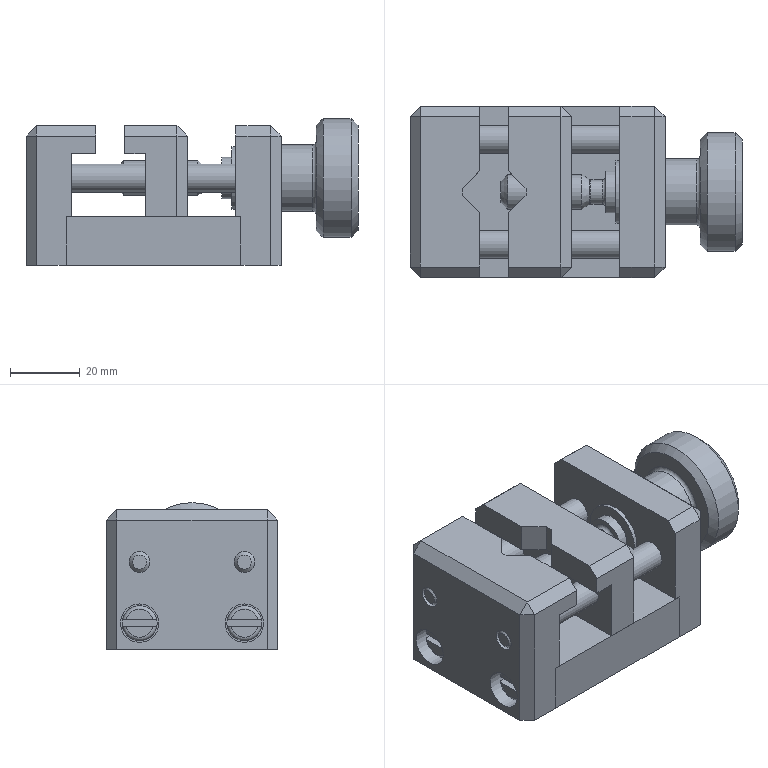Assembly | NX | mm | 13 component files | 13 solids | 208 faces | box 95 x 49 x 42 mm | volume 117232 mm3 | plane 112 | cylinder 50 | cone 27 | torus 19 | commonest cylinder face diameters 6 x16 10 x6 5.8 x4 8 x4 6.6 x4 11 x4 4 x3 12 x3
Bill of materials:
unnamed part 1 | 1 |  | Plain solid cylindrical pin with a small chamfer at both ends.
unnamed part 2 | 1 |  | Thick rectangular plate or block with four round through-holes in a 2x2 pattern, chamfered upper corners, a stepped profile, a V-shaped notch on one side face, and a rectangular step/notch feature at the top edge.
unnamed part 3 | 2 |  | Stepped cylindrical shaft: a larger-diameter central body with smaller-diameter journals at both ends, each end chamfered.
unnamed part 4 | 1 |  | Rectangular block with three round blind holes in a row on one side face; the middle hole is smaller than the two outer holes.
unnamed part 5 | 1 |  | Block with a stepped (L/T-like) cross-section, chamfered top edges, three round through-holes in a row (center hole larger), and a V-shaped notch on one end face.
unnamed part 6 | 1 |  | Rectangular plate with chamfered top edges, a small step on one face, and seven round through-holes of varying size: one large center hole, four medium holes near the corners, and a small hole at the lower center.
unnamed part 7 | 4 |  | Headed cylindrical fastener-like part: a short cylindrical head with rounded outer edge and a straight slot across its end, and a plain cylindrical shank with a chamfered tip.
unnamed part 8 | 1 |  | Thin flat annular ring (washer-like) with a plain circular inner bore and outer edge.
unnamed part 9 | 1 |  | Stepped turned pin with a large chamfered disc head, an intermediate-diameter collar, a reduced shank section with small grooves, a narrow neck, and a chamfered cylindrical tip.
Mates:
1. fix | base_plate 1 component
2. concentric | fixed_bracket 1 edge | base_plate 1 edge
3. parallel | fixed_bracket 1 face | base_plate 1 face
4. concentric | fixed_jaw 1 edge | base_plate 1 edge
5. parallel | fixed_jaw 1 face | base_plate 1 face
6. concentric | leadscrew 1 edge | fixed_bracket 1 edge
7. touch align | movable_jaw 1 face | leadscrew 1 face
8. parallel | movable_jaw 1 face | fixed_bracket 1 face
9. concentric | dowel_pin 1 edge | fixed_bracket 1 edge
10. concentric | sliding_guide 2 edge | fixed_bracket 1 edge
11. concentric | sliding_guide 1 edge | fixed_bracket 1 edge
12. concentric | slotted_cap_screw 4 edge | fixed_bracket 1 edge
13. concentric | fixed_bracket 1 edge | slotted_cap_screw 3 edge
14. concentric | slotted_cap_screw 2 edge | fixed_jaw 1 edge
15. concentric | slotted_cap_screw 1 edge | fixed_jaw 1 edge
16. concentric | retaining_ring 1 arc | leadscrew 1 edge